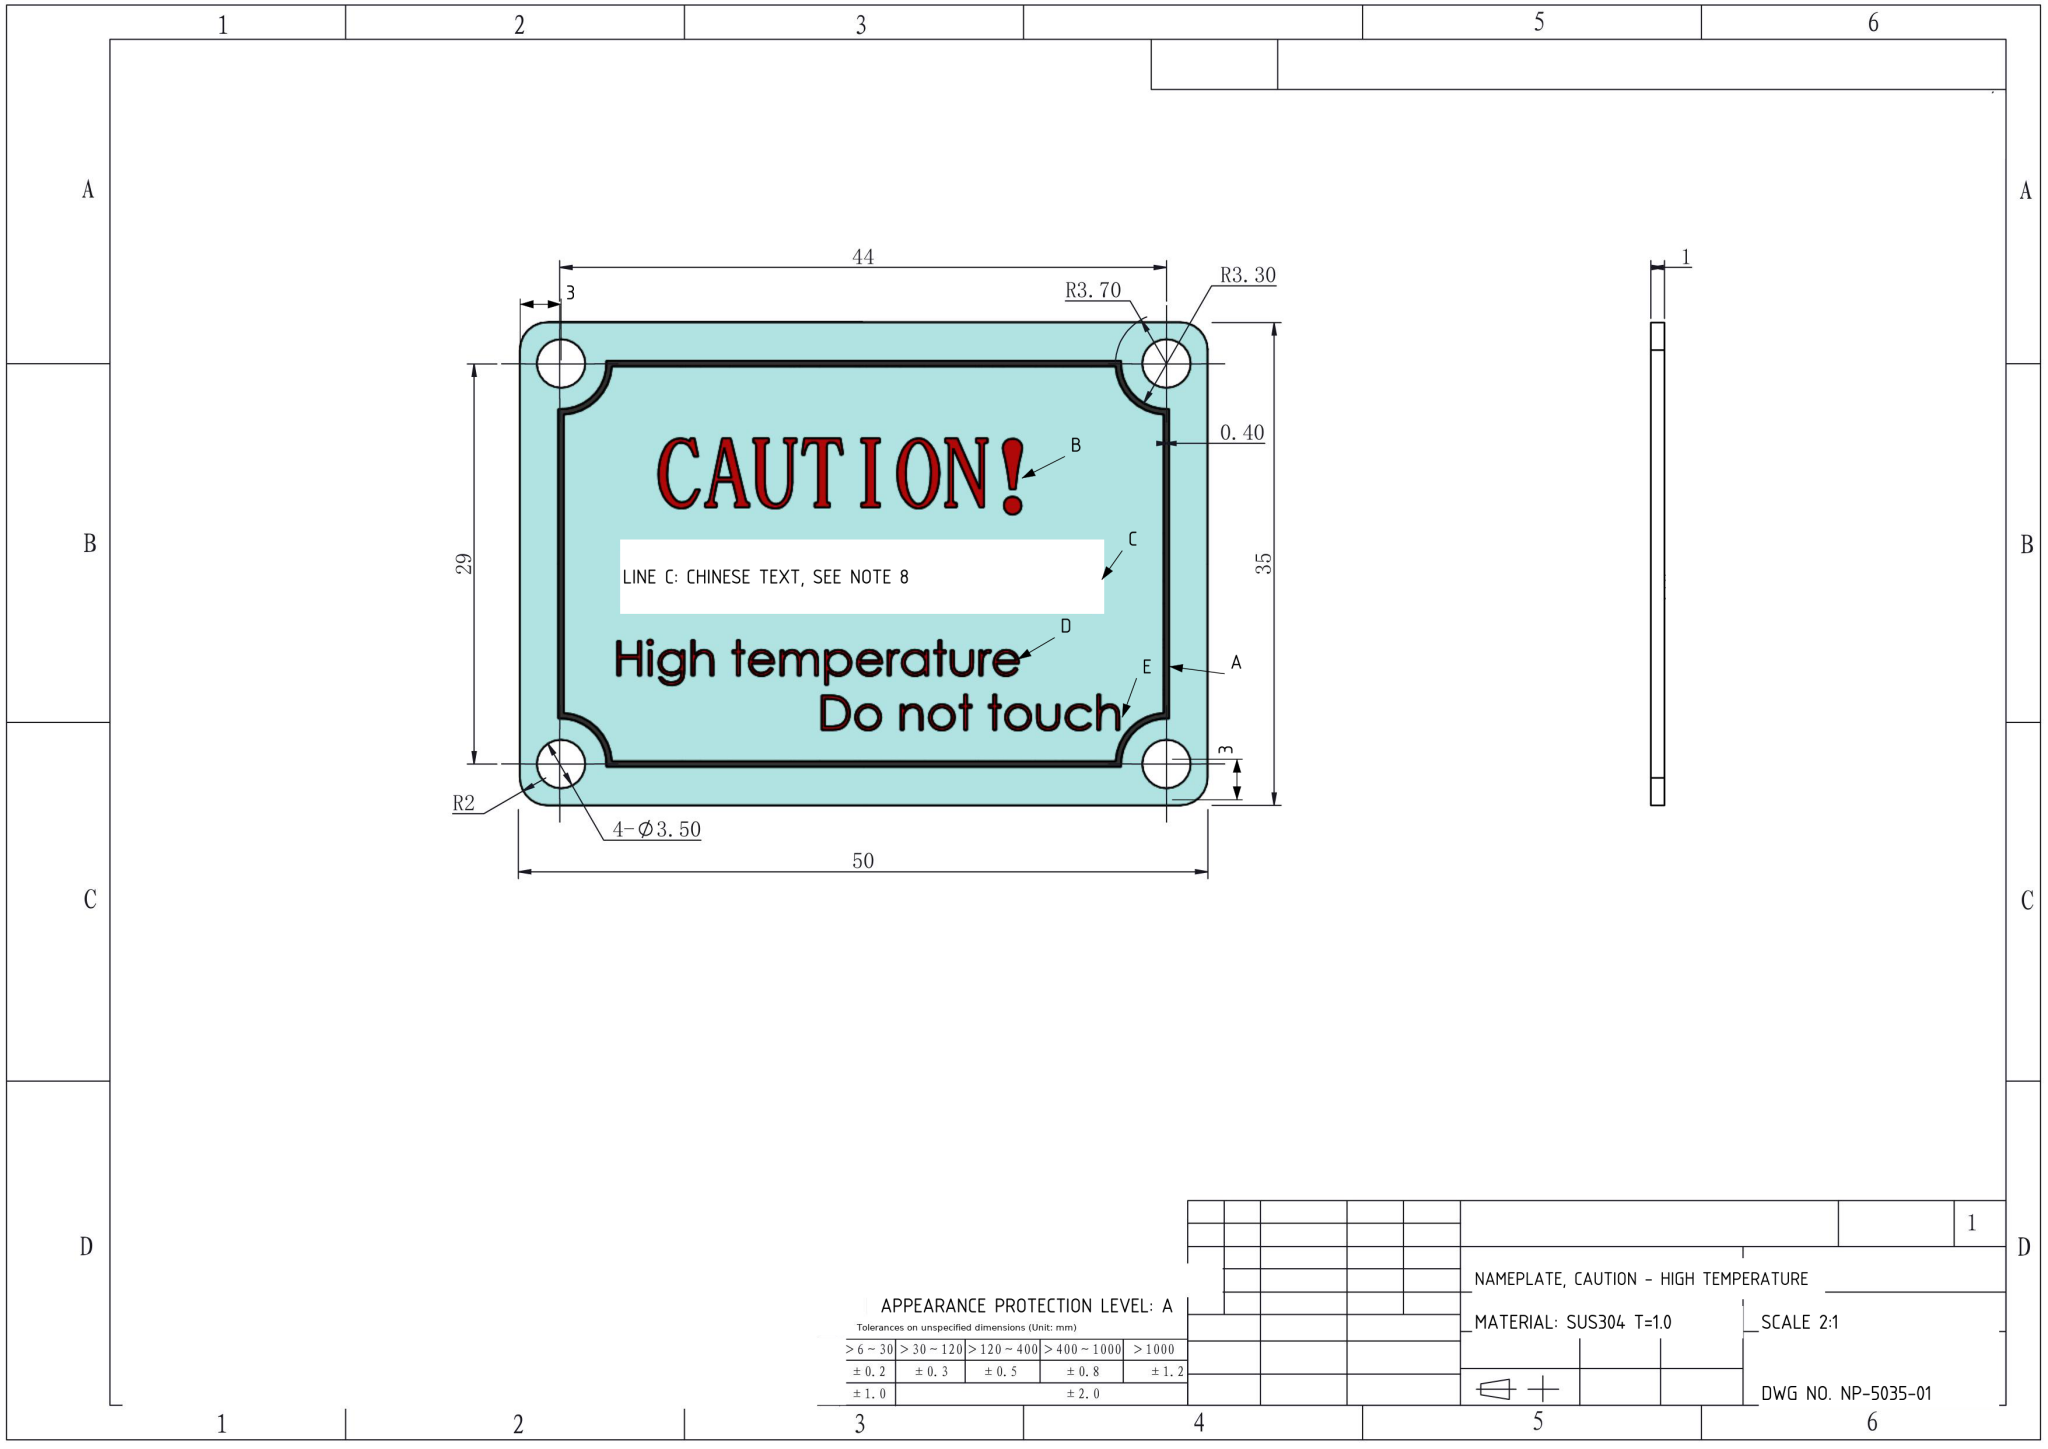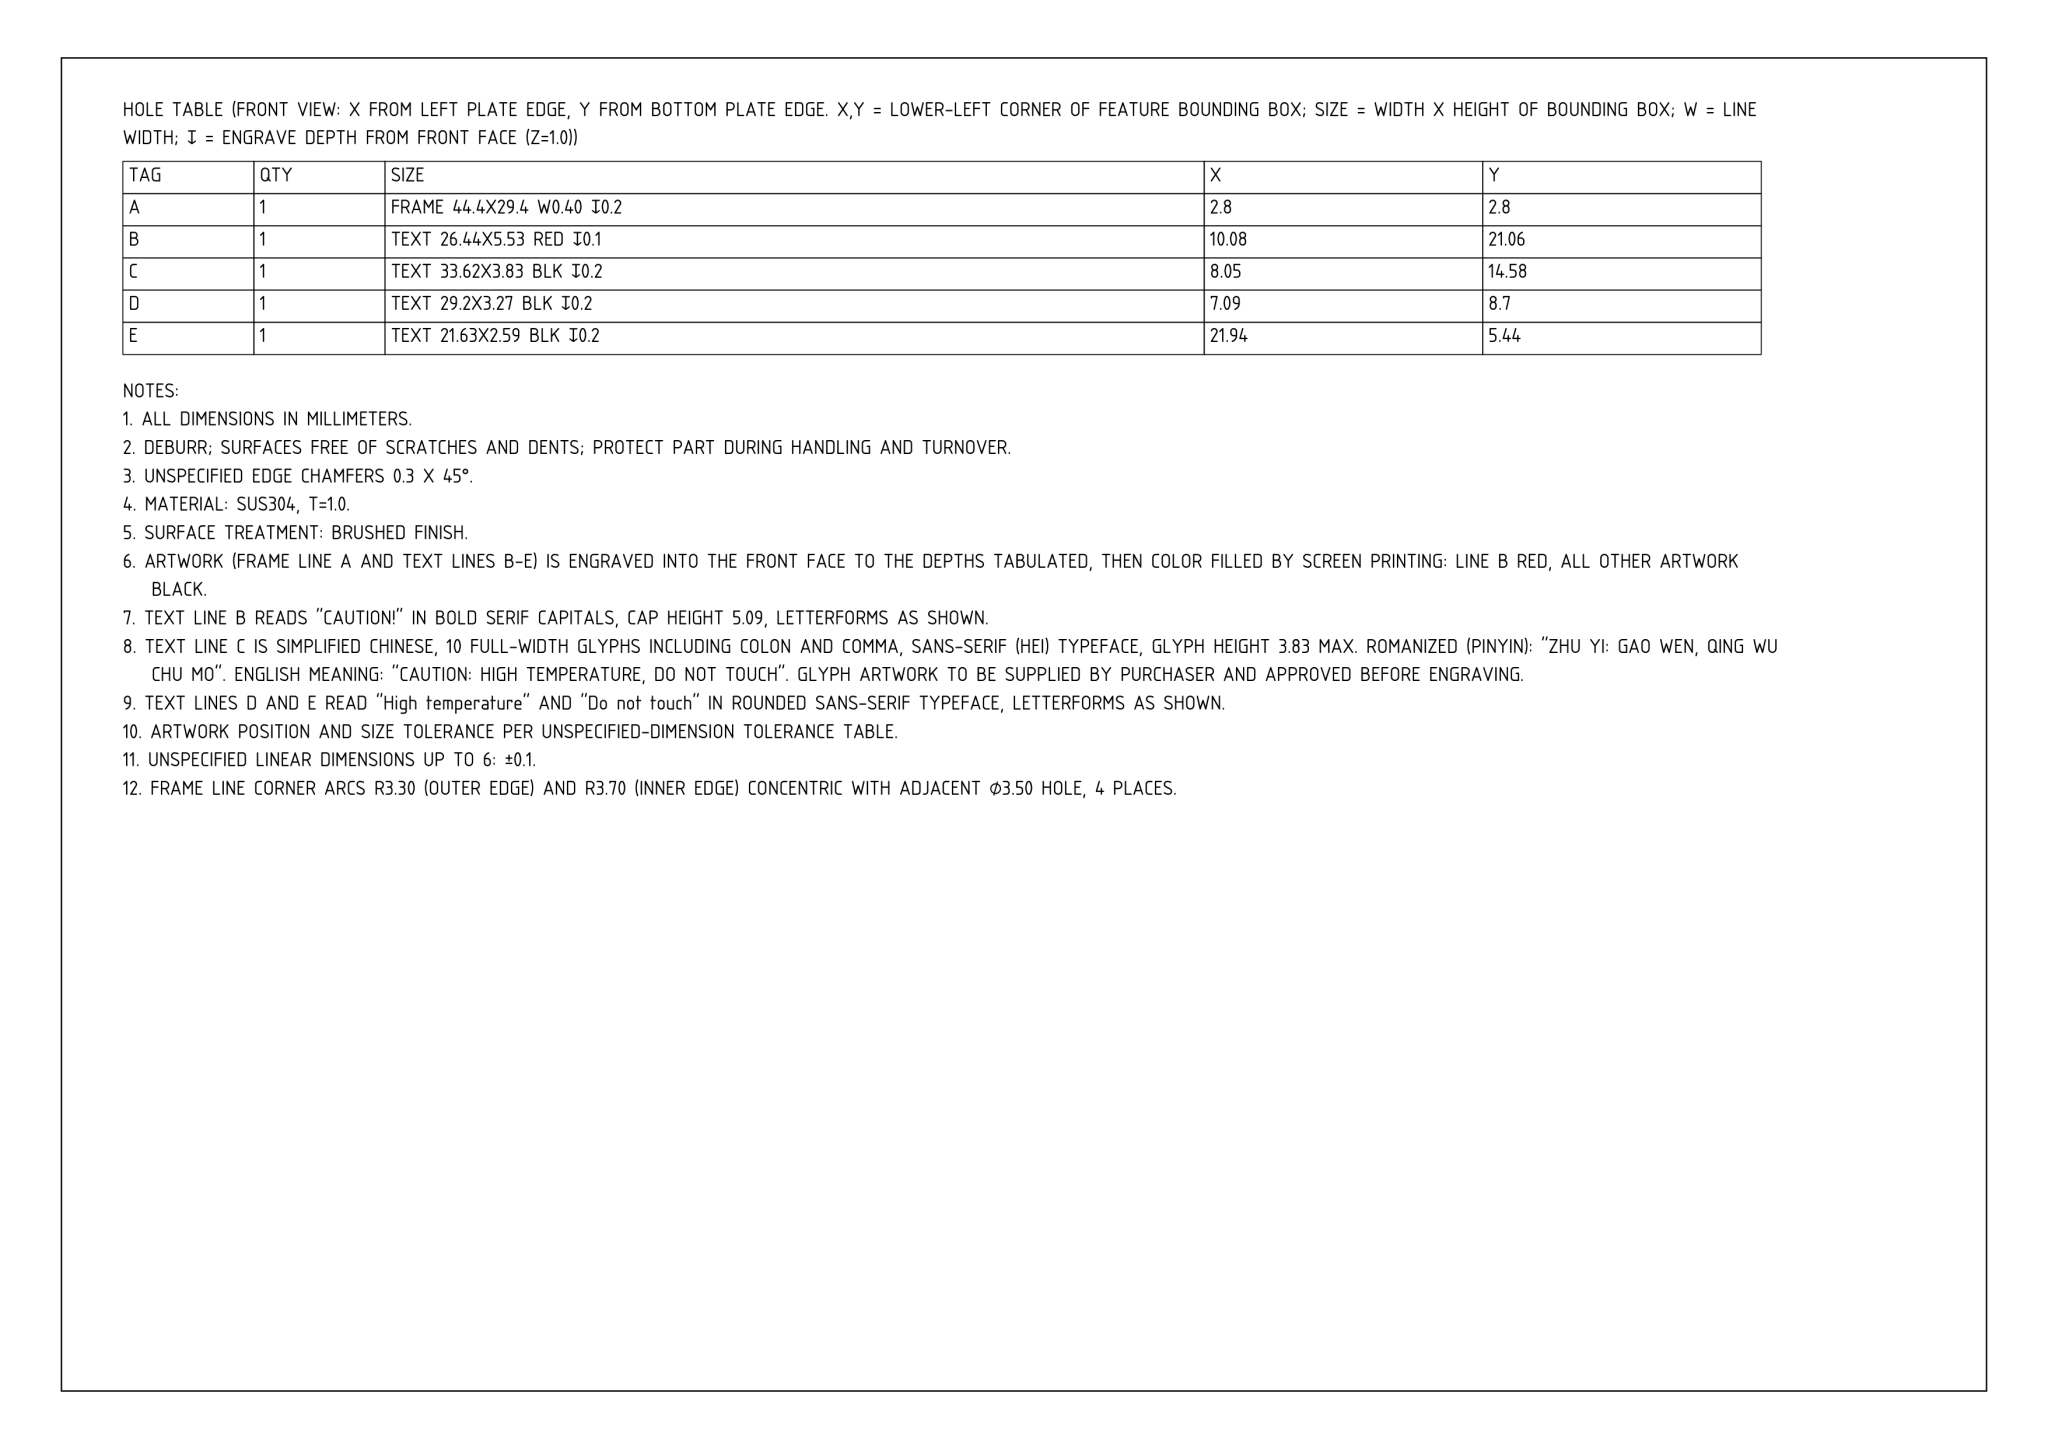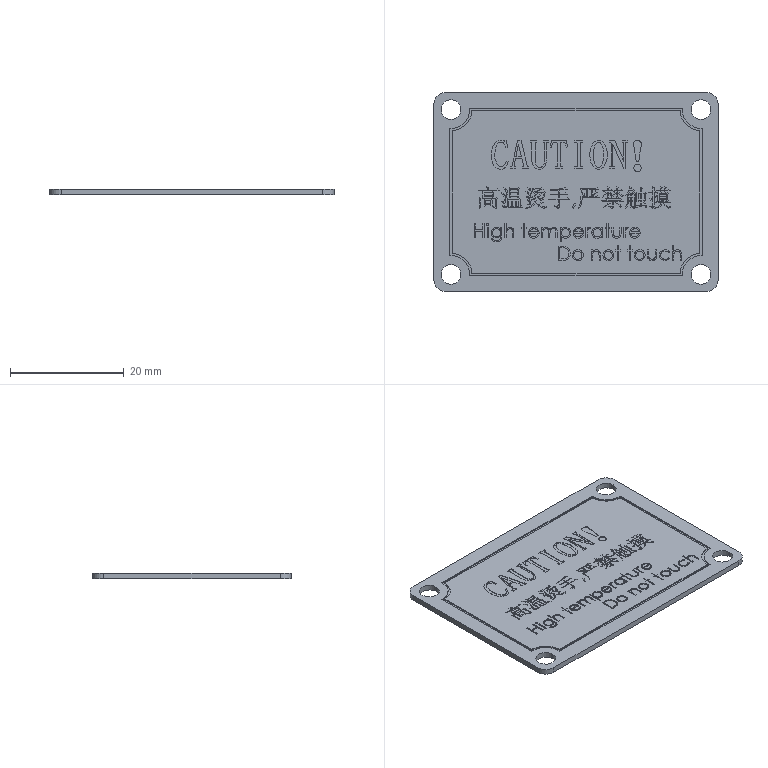Part | NX | mm | 1 solid | 1090 faces | box 50 x 35 x 1 mm | volume 1682 mm3 | plane 689 | spline 379 | cylinder 22 | commonest cylinder face diameters 3.5 x8 6.6 x6 7.4 x4 4 x4